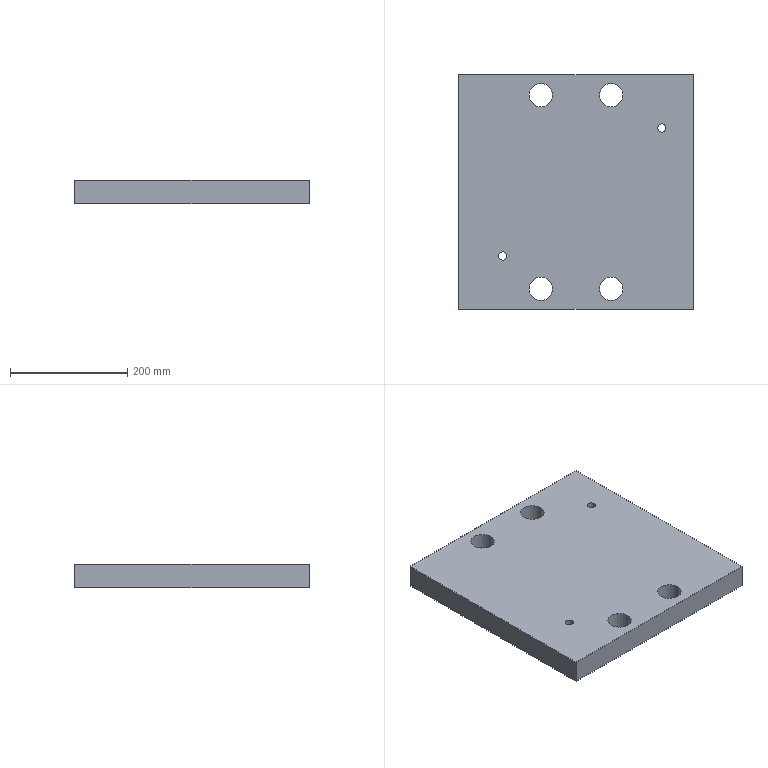Component | NX | LOCATING_BASE_PLATE | 1 solid | 12 faces | box 400 x 400 x 40 mm | volume 6186623 mm3 | plane 6 | cylinder 6 | commonest cylinder face diameters 40 x4 14 x2
STEP:
#1=CARTESIAN_POINT('',(0.,0.,0.));
#2=DIRECTION('',(0.,0.,1.));
#3=DIRECTION('',(1.,0.,0.));
#4=AXIS2_PLACEMENT_3D('',#1,#2,#3);
#5=CARTESIAN_POINT('',(-40.,165.,90.));
#6=VERTEX_POINT('',#5);
#7=CARTESIAN_POINT('',(-60.,165.,90.));
#8=DIRECTION('',(0.,0.,-1.));
#9=DIRECTION('',(1.,0.,0.));
#10=AXIS2_PLACEMENT_3D('',#7,#8,#9);
#11=CIRCLE('',#10,20.);
#12=CARTESIAN_POINT('',(0.,-0.,90.));
#13=DIRECTION('',(0.,0.,1.));
#14=DIRECTION('',(1.,0.,0.));
#15=AXIS2_PLACEMENT_3D('',#12,#13,#14);
#16=PLANE('',#15);
#17=CARTESIAN_POINT('',(-40.,165.));
#18=CARTESIAN_POINT('',(-40.,130.359));
#19=CARTESIAN_POINT('',(-70.,147.679));
#20=CARTESIAN_POINT('',(-100.,165.));
#21=CARTESIAN_POINT('',(-70.,182.321));
#22=CARTESIAN_POINT('',(-40.,199.641));
#23=CARTESIAN_POINT('',(-40.,165.));
#24=(BOUNDED_CURVE()B_SPLINE_CURVE(2,(#17,#18,#19,#20,#21,#22,#23),.UNSPECIFIED.,.T.,.F.)B_SPLINE_CURVE_WITH_KNOTS((1,2,2,2,2,1),(-2.094,0.,2.094,4.189,6.283,8.378),.UNSPECIFIED.)CURVE()GEOMETRIC_REPRESENTATION_ITEM()RATIONAL_B_SPLINE_CURVE((1.,0.5,1.,0.5,1.,0.5,1.))REPRESENTATION_ITEM(''));
#25=(GEOMETRIC_REPRESENTATION_CONTEXT(2)PARAMETRIC_REPRESENTATION_CONTEXT()REPRESENTATION_CONTEXT('',''));
#26=DEFINITIONAL_REPRESENTATION('',(#24),#25);
#27=PCURVE('',#16,#26);
#28=CARTESIAN_POINT('',(-60.,165.,40.));
#29=DIRECTION('',(0.,0.,1.));
#30=DIRECTION('',(1.,0.,0.));
#31=AXIS2_PLACEMENT_3D('',#28,#29,#30);
#32=CYLINDRICAL_SURFACE('',#31,20.);
#33=CARTESIAN_POINT('',(6.283,50.));
#34=DIRECTION('',(-1.,0.));
#35=VECTOR('',#34,1.);
#36=LINE('',#33,#35);
#37=(GEOMETRIC_REPRESENTATION_CONTEXT(2)PARAMETRIC_REPRESENTATION_CONTEXT()REPRESENTATION_CONTEXT('',''));
#38=DEFINITIONAL_REPRESENTATION('',(#36),#37);
#39=PCURVE('',#32,#38);
#40=SURFACE_CURVE('',#11,(#27,#39),.PCURVE_S1.);
#41=EDGE_CURVE('',#6,#6,#40,.T.);
#42=ORIENTED_EDGE('',*,*,#41,.T.);
#43=EDGE_LOOP('',(#42));
#44=FACE_BOUND('',#43,.T.);
#45=CARTESIAN_POINT('',(40.,165.,90.));
#46=VERTEX_POINT('',#45);
#47=CARTESIAN_POINT('',(80.,165.,90.));
#48=VERTEX_POINT('',#47);
#49=CARTESIAN_POINT('',(60.,165.,90.));
#50=DIRECTION('',(0.,0.,1.));
#51=DIRECTION('',(-1.,0.,0.));
#52=AXIS2_PLACEMENT_3D('',#49,#50,#51);
#53=CIRCLE('',#52,20.);
#54=CARTESIAN_POINT('',(60.,165.));
#55=DIRECTION('',(-1.,0.));
#56=AXIS2_PLACEMENT_2D('',#54,#55);
#57=CIRCLE('',#56,20.);
#58=(GEOMETRIC_REPRESENTATION_CONTEXT(2)PARAMETRIC_REPRESENTATION_CONTEXT()REPRESENTATION_CONTEXT('',''));
#59=DEFINITIONAL_REPRESENTATION('',(#57),#58);
#60=PCURVE('',#16,#59);
#61=CARTESIAN_POINT('',(60.,165.,40.));
#62=DIRECTION('',(0.,0.,1.));
#63=DIRECTION('',(1.,0.,0.));
#64=AXIS2_PLACEMENT_3D('',#61,#62,#63);
#65=CYLINDRICAL_SURFACE('',#64,20.);
#66=CARTESIAN_POINT('',(3.142,50.));
#67=DIRECTION('',(1.,0.));
#68=VECTOR('',#67,1.);
#69=LINE('',#66,#68);
#70=(GEOMETRIC_REPRESENTATION_CONTEXT(2)PARAMETRIC_REPRESENTATION_CONTEXT()REPRESENTATION_CONTEXT('',''));
#71=DEFINITIONAL_REPRESENTATION('',(#69),#70);
#72=PCURVE('',#65,#71);
#73=SURFACE_CURVE('',#53,(#60,#72),.PCURVE_S1.);
#74=EDGE_CURVE('',#46,#48,#73,.T.);
#75=ORIENTED_EDGE('',*,*,#74,.F.);
#76=CARTESIAN_POINT('',(60.,165.,90.));
#77=DIRECTION('',(0.,0.,1.));
#78=DIRECTION('',(-1.,0.,0.));
#79=AXIS2_PLACEMENT_3D('',#76,#77,#78);
#80=CIRCLE('',#79,20.);
#81=CARTESIAN_POINT('',(60.,165.));
#82=DIRECTION('',(-1.,0.));
#83=AXIS2_PLACEMENT_2D('',#81,#82);
#84=CIRCLE('',#83,20.);
#85=(GEOMETRIC_REPRESENTATION_CONTEXT(2)PARAMETRIC_REPRESENTATION_CONTEXT()REPRESENTATION_CONTEXT('',''));
#86=DEFINITIONAL_REPRESENTATION('',(#84),#85);
#87=PCURVE('',#16,#86);
#88=CARTESIAN_POINT('',(-3.142,50.));
#89=DIRECTION('',(1.,0.));
#90=VECTOR('',#89,1.);
#91=LINE('',#88,#90);
#92=(GEOMETRIC_REPRESENTATION_CONTEXT(2)PARAMETRIC_REPRESENTATION_CONTEXT()REPRESENTATION_CONTEXT('',''));
#93=DEFINITIONAL_REPRESENTATION('',(#91),#92);
#94=PCURVE('',#65,#93);
#95=SURFACE_CURVE('',#80,(#87,#94),.PCURVE_S1.);
#96=EDGE_CURVE('',#48,#46,#95,.T.);
#97=ORIENTED_EDGE('',*,*,#96,.F.);
#98=EDGE_LOOP('',(#75,#97));
#99=FACE_BOUND('',#98,.T.);
#100=CARTESIAN_POINT('',(153.,109.,90.));
#101=VERTEX_POINT('',#100);
#102=CARTESIAN_POINT('',(146.,109.,90.));
#103=DIRECTION('',(0.,0.,1.));
#104=DIRECTION('',(1.,0.,0.));
#105=AXIS2_PLACEMENT_3D('',#102,#103,#104);
#106=CIRCLE('',#105,7.);
#107=CARTESIAN_POINT('',(146.,109.));
#108=DIRECTION('',(1.,0.));
#109=AXIS2_PLACEMENT_2D('',#107,#108);
#110=CIRCLE('',#109,7.);
#111=(GEOMETRIC_REPRESENTATION_CONTEXT(2)PARAMETRIC_REPRESENTATION_CONTEXT()REPRESENTATION_CONTEXT('',''));
#112=DEFINITIONAL_REPRESENTATION('',(#110),#111);
#113=PCURVE('',#16,#112);
#114=CARTESIAN_POINT('',(146.,109.,50.));
#115=DIRECTION('',(0.,0.,1.));
#116=DIRECTION('',(1.,0.,0.));
#117=AXIS2_PLACEMENT_3D('',#114,#115,#116);
#118=CYLINDRICAL_SURFACE('',#117,7.);
#119=CARTESIAN_POINT('',(0.,40.));
#120=DIRECTION('',(1.,0.));
#121=VECTOR('',#120,1.);
#122=LINE('',#119,#121);
#123=(GEOMETRIC_REPRESENTATION_CONTEXT(2)PARAMETRIC_REPRESENTATION_CONTEXT()REPRESENTATION_CONTEXT('',''));
#124=DEFINITIONAL_REPRESENTATION('',(#122),#123);
#125=PCURVE('',#118,#124);
#126=SURFACE_CURVE('',#106,(#113,#125),.PCURVE_S1.);
#127=EDGE_CURVE('',#101,#101,#126,.T.);
#128=ORIENTED_EDGE('',*,*,#127,.F.);
#129=EDGE_LOOP('',(#128));
#130=FACE_BOUND('',#129,.T.);
#131=CARTESIAN_POINT('',(-118.,-109.,90.));
#132=VERTEX_POINT('',#131);
#133=CARTESIAN_POINT('',(-125.,-109.,90.));
#134=DIRECTION('',(0.,0.,1.));
#135=DIRECTION('',(1.,0.,0.));
#136=AXIS2_PLACEMENT_3D('',#133,#134,#135);
#137=CIRCLE('',#136,7.);
#138=CARTESIAN_POINT('',(-125.,-109.));
#139=DIRECTION('',(1.,0.));
#140=AXIS2_PLACEMENT_2D('',#138,#139);
#141=CIRCLE('',#140,7.);
#142=(GEOMETRIC_REPRESENTATION_CONTEXT(2)PARAMETRIC_REPRESENTATION_CONTEXT()REPRESENTATION_CONTEXT('',''));
#143=DEFINITIONAL_REPRESENTATION('',(#141),#142);
#144=PCURVE('',#16,#143);
#145=CARTESIAN_POINT('',(-125.,-109.,50.));
#146=DIRECTION('',(0.,0.,1.));
#147=DIRECTION('',(1.,0.,0.));
#148=AXIS2_PLACEMENT_3D('',#145,#146,#147);
#149=CYLINDRICAL_SURFACE('',#148,7.);
#150=CARTESIAN_POINT('',(0.,40.));
#151=DIRECTION('',(1.,0.));
#152=VECTOR('',#151,1.);
#153=LINE('',#150,#152);
#154=(GEOMETRIC_REPRESENTATION_CONTEXT(2)PARAMETRIC_REPRESENTATION_CONTEXT()REPRESENTATION_CONTEXT('',''));
#155=DEFINITIONAL_REPRESENTATION('',(#153),#154);
#156=PCURVE('',#149,#155);
#157=SURFACE_CURVE('',#137,(#144,#156),.PCURVE_S1.);
#158=EDGE_CURVE('',#132,#132,#157,.T.);
#159=ORIENTED_EDGE('',*,*,#158,.F.);
#160=EDGE_LOOP('',(#159));
#161=FACE_BOUND('',#160,.T.);
#162=CARTESIAN_POINT('',(-200.,200.,90.));
#163=VERTEX_POINT('',#162);
#164=CARTESIAN_POINT('',(-200.,-200.,90.));
#165=VERTEX_POINT('',#164);
#166=CARTESIAN_POINT('',(-200.,200.,90.));
#167=DIRECTION('',(0.,-1.,0.));
#168=VECTOR('',#167,1.);
#169=LINE('',#166,#168);
#170=CARTESIAN_POINT('',(-200.,200.));
#171=DIRECTION('',(0.,-1.));
#172=VECTOR('',#171,1.);
#173=LINE('',#170,#172);
#174=(GEOMETRIC_REPRESENTATION_CONTEXT(2)PARAMETRIC_REPRESENTATION_CONTEXT()REPRESENTATION_CONTEXT('',''));
#175=DEFINITIONAL_REPRESENTATION('',(#173),#174);
#176=PCURVE('',#16,#175);
#177=CARTESIAN_POINT('',(-200.,200.,90.));
#178=DIRECTION('',(1.,0.,0.));
#179=DIRECTION('',(0.,0.,-1.));
#180=AXIS2_PLACEMENT_3D('',#177,#178,#179);
#181=PLANE('',#180);
#182=CARTESIAN_POINT('',(0.,0.));
#183=DIRECTION('',(0.,-1.));
#184=VECTOR('',#183,1.);
#185=LINE('',#182,#184);
#186=(GEOMETRIC_REPRESENTATION_CONTEXT(2)PARAMETRIC_REPRESENTATION_CONTEXT()REPRESENTATION_CONTEXT('',''));
#187=DEFINITIONAL_REPRESENTATION('',(#185),#186);
#188=PCURVE('',#181,#187);
#189=SURFACE_CURVE('',#169,(#176,#188),.PCURVE_S1.);
#190=EDGE_CURVE('',#163,#165,#189,.T.);
#191=ORIENTED_EDGE('',*,*,#190,.T.);
#192=CARTESIAN_POINT('',(200.,-200.,90.));
#193=VERTEX_POINT('',#192);
#194=CARTESIAN_POINT('',(-200.,-200.,90.));
#195=DIRECTION('',(1.,0.,0.));
#196=VECTOR('',#195,1.);
#197=LINE('',#194,#196);
#198=CARTESIAN_POINT('',(-200.,-200.));
#199=DIRECTION('',(1.,0.));
#200=VECTOR('',#199,1.);
#201=LINE('',#198,#200);
#202=(GEOMETRIC_REPRESENTATION_CONTEXT(2)PARAMETRIC_REPRESENTATION_CONTEXT()REPRESENTATION_CONTEXT('',''));
#203=DEFINITIONAL_REPRESENTATION('',(#201),#202);
#204=PCURVE('',#16,#203);
#205=CARTESIAN_POINT('',(-200.,-200.,90.));
#206=DIRECTION('',(0.,1.,0.));
#207=DIRECTION('',(0.,0.,1.));
#208=AXIS2_PLACEMENT_3D('',#205,#206,#207);
#209=PLANE('',#208);
#210=CARTESIAN_POINT('',(0.,0.));
#211=DIRECTION('',(0.,1.));
#212=VECTOR('',#211,1.);
#213=LINE('',#210,#212);
#214=(GEOMETRIC_REPRESENTATION_CONTEXT(2)PARAMETRIC_REPRESENTATION_CONTEXT()REPRESENTATION_CONTEXT('',''));
#215=DEFINITIONAL_REPRESENTATION('',(#213),#214);
#216=PCURVE('',#209,#215);
#217=SURFACE_CURVE('',#197,(#204,#216),.PCURVE_S1.);
#218=EDGE_CURVE('',#165,#193,#217,.T.);
#219=ORIENTED_EDGE('',*,*,#218,.T.);
#220=CARTESIAN_POINT('',(200.,200.,90.));
#221=VERTEX_POINT('',#220);
#222=CARTESIAN_POINT('',(200.,-200.,90.));
#223=DIRECTION('',(0.,1.,0.));
#224=VECTOR('',#223,1.);
#225=LINE('',#222,#224);
#226=CARTESIAN_POINT('',(200.,-200.));
#227=DIRECTION('',(0.,1.));
#228=VECTOR('',#227,1.);
#229=LINE('',#226,#228);
#230=(GEOMETRIC_REPRESENTATION_CONTEXT(2)PARAMETRIC_REPRESENTATION_CONTEXT()REPRESENTATION_CONTEXT('',''));
#231=DEFINITIONAL_REPRESENTATION('',(#229),#230);
#232=PCURVE('',#16,#231);
#233=CARTESIAN_POINT('',(200.,-200.,90.));
#234=DIRECTION('',(-1.,0.,0.));
#235=DIRECTION('',(0.,0.,1.));
#236=AXIS2_PLACEMENT_3D('',#233,#234,#235);
#237=PLANE('',#236);
#238=CARTESIAN_POINT('',(0.,0.));
#239=DIRECTION('',(0.,1.));
#240=VECTOR('',#239,1.);
#241=LINE('',#238,#240);
#242=(GEOMETRIC_REPRESENTATION_CONTEXT(2)PARAMETRIC_REPRESENTATION_CONTEXT()REPRESENTATION_CONTEXT('',''));
#243=DEFINITIONAL_REPRESENTATION('',(#241),#242);
#244=PCURVE('',#237,#243);
#245=SURFACE_CURVE('',#225,(#232,#244),.PCURVE_S1.);
#246=EDGE_CURVE('',#193,#221,#245,.T.);
#247=ORIENTED_EDGE('',*,*,#246,.T.);
#248=CARTESIAN_POINT('',(200.,200.,90.));
#249=DIRECTION('',(-1.,0.,0.));
#250=VECTOR('',#249,1.);
#251=LINE('',#248,#250);
#252=CARTESIAN_POINT('',(200.,200.));
#253=DIRECTION('',(-1.,0.));
#254=VECTOR('',#253,1.);
#255=LINE('',#252,#254);
#256=(GEOMETRIC_REPRESENTATION_CONTEXT(2)PARAMETRIC_REPRESENTATION_CONTEXT()REPRESENTATION_CONTEXT('',''));
#257=DEFINITIONAL_REPRESENTATION('',(#255),#256);
#258=PCURVE('',#16,#257);
#259=CARTESIAN_POINT('',(200.,200.,90.));
#260=DIRECTION('',(0.,-1.,0.));
#261=DIRECTION('',(0.,0.,-1.));
#262=AXIS2_PLACEMENT_3D('',#259,#260,#261);
#263=PLANE('',#262);
#264=CARTESIAN_POINT('',(0.,0.));
#265=DIRECTION('',(0.,-1.));
#266=VECTOR('',#265,1.);
#267=LINE('',#264,#266);
#268=(GEOMETRIC_REPRESENTATION_CONTEXT(2)PARAMETRIC_REPRESENTATION_CONTEXT()REPRESENTATION_CONTEXT('',''));
#269=DEFINITIONAL_REPRESENTATION('',(#267),#268);
#270=PCURVE('',#263,#269);
#271=SURFACE_CURVE('',#251,(#258,#270),.PCURVE_S1.);
#272=EDGE_CURVE('',#221,#163,#271,.T.);
#273=ORIENTED_EDGE('',*,*,#272,.T.);
#274=EDGE_LOOP('',(#191,#219,#247,#273));
#275=FACE_BOUND('',#274,.T.);
#276=CARTESIAN_POINT('',(-40.,-165.,90.));
#277=VERTEX_POINT('',#276);
#278=CARTESIAN_POINT('',(-60.,-165.,90.));
#279=DIRECTION('',(0.,0.,1.));
#280=DIRECTION('',(1.,0.,0.));
#281=AXIS2_PLACEMENT_3D('',#278,#279,#280);
#282=CIRCLE('',#281,20.);
#283=CARTESIAN_POINT('',(-60.,-165.));
#284=DIRECTION('',(1.,0.));
#285=AXIS2_PLACEMENT_2D('',#283,#284);
#286=CIRCLE('',#285,20.);
#287=(GEOMETRIC_REPRESENTATION_CONTEXT(2)PARAMETRIC_REPRESENTATION_CONTEXT()REPRESENTATION_CONTEXT('',''));
#288=DEFINITIONAL_REPRESENTATION('',(#286),#287);
#289=PCURVE('',#16,#288);
#290=CARTESIAN_POINT('',(-60.,-165.,40.));
#291=DIRECTION('',(0.,0.,1.));
#292=DIRECTION('',(1.,0.,0.));
#293=AXIS2_PLACEMENT_3D('',#290,#291,#292);
#294=CYLINDRICAL_SURFACE('',#293,20.);
#295=CARTESIAN_POINT('',(0.,50.));
#296=DIRECTION('',(1.,0.));
#297=VECTOR('',#296,1.);
#298=LINE('',#295,#297);
#299=(GEOMETRIC_REPRESENTATION_CONTEXT(2)PARAMETRIC_REPRESENTATION_CONTEXT()REPRESENTATION_CONTEXT('',''));
#300=DEFINITIONAL_REPRESENTATION('',(#298),#299);
#301=PCURVE('',#294,#300);
#302=SURFACE_CURVE('',#282,(#289,#301),.PCURVE_S1.);
#303=EDGE_CURVE('',#277,#277,#302,.T.);
#304=ORIENTED_EDGE('',*,*,#303,.F.);
#305=EDGE_LOOP('',(#304));
#306=FACE_BOUND('',#305,.T.);
#307=CARTESIAN_POINT('',(40.,-165.,90.));
#308=VERTEX_POINT('',#307);
#309=CARTESIAN_POINT('',(80.,-165.,90.));
#310=VERTEX_POINT('',#309);
#311=CARTESIAN_POINT('',(60.,-165.,90.));
#312=DIRECTION('',(0.,0.,-1.));
#313=DIRECTION('',(-1.,0.,0.));
#314=AXIS2_PLACEMENT_3D('',#311,#312,#313);
#315=CIRCLE('',#314,20.);
#316=CARTESIAN_POINT('',(40.,-165.));
#317=CARTESIAN_POINT('',(40.,-130.359));
#318=CARTESIAN_POINT('',(70.,-147.679));
#319=CARTESIAN_POINT('',(100.,-165.));
#320=CARTESIAN_POINT('',(70.,-182.321));
#321=CARTESIAN_POINT('',(40.,-199.641));
#322=CARTESIAN_POINT('',(40.,-165.));
#323=(BOUNDED_CURVE()B_SPLINE_CURVE(2,(#316,#317,#318,#319,#320,#321,#322),.UNSPECIFIED.,.T.,.F.)B_SPLINE_CURVE_WITH_KNOTS((1,2,2,2,2,1),(-2.094,0.,2.094,4.189,6.283,8.378),.UNSPECIFIED.)CURVE()GEOMETRIC_REPRESENTATION_ITEM()RATIONAL_B_SPLINE_CURVE((1.,0.5,1.,0.5,1.,0.5,1.))REPRESENTATION_ITEM(''));
#324=(GEOMETRIC_REPRESENTATION_CONTEXT(2)PARAMETRIC_REPRESENTATION_CONTEXT()REPRESENTATION_CONTEXT('',''));
#325=DEFINITIONAL_REPRESENTATION('',(#323),#324);
#326=PCURVE('',#16,#325);
#327=CARTESIAN_POINT('',(60.,-165.,40.));
#328=DIRECTION('',(0.,0.,1.));
#329=DIRECTION('',(1.,0.,0.));
#330=AXIS2_PLACEMENT_3D('',#327,#328,#329);
#331=CYLINDRICAL_SURFACE('',#330,20.);
#332=CARTESIAN_POINT('',(3.142,50.));
#333=DIRECTION('',(-1.,0.));
#334=VECTOR('',#333,1.);
#335=LINE('',#332,#334);
#336=(GEOMETRIC_REPRESENTATION_CONTEXT(2)PARAMETRIC_REPRESENTATION_CONTEXT()REPRESENTATION_CONTEXT('',''));
#337=DEFINITIONAL_REPRESENTATION('',(#335),#336);
#338=PCURVE('',#331,#337);
#339=SURFACE_CURVE('',#315,(#326,#338),.PCURVE_S1.);
#340=EDGE_CURVE('',#308,#310,#339,.T.);
#341=ORIENTED_EDGE('',*,*,#340,.T.);
#342=CARTESIAN_POINT('',(60.,-165.,90.));
#343=DIRECTION('',(0.,0.,-1.));
#344=DIRECTION('',(-1.,0.,0.));
#345=AXIS2_PLACEMENT_3D('',#342,#343,#344);
#346=CIRCLE('',#345,20.);
#347=CARTESIAN_POINT('',(40.,-165.));
#348=CARTESIAN_POINT('',(40.,-130.359));
#349=CARTESIAN_POINT('',(70.,-147.679));
#350=CARTESIAN_POINT('',(100.,-165.));
#351=CARTESIAN_POINT('',(70.,-182.321));
#352=CARTESIAN_POINT('',(40.,-199.641));
#353=CARTESIAN_POINT('',(40.,-165.));
#354=(BOUNDED_CURVE()B_SPLINE_CURVE(2,(#347,#348,#349,#350,#351,#352,#353),.UNSPECIFIED.,.T.,.F.)B_SPLINE_CURVE_WITH_KNOTS((1,2,2,2,2,1),(-2.094,0.,2.094,4.189,6.283,8.378),.UNSPECIFIED.)CURVE()GEOMETRIC_REPRESENTATION_ITEM()RATIONAL_B_SPLINE_CURVE((1.,0.5,1.,0.5,1.,0.5,1.))REPRESENTATION_ITEM(''));
#355=(GEOMETRIC_REPRESENTATION_CONTEXT(2)PARAMETRIC_REPRESENTATION_CONTEXT()REPRESENTATION_CONTEXT('',''));
#356=DEFINITIONAL_REPRESENTATION('',(#354),#355);
#357=PCURVE('',#16,#356);
#358=CARTESIAN_POINT('',(9.425,50.));
#359=DIRECTION('',(-1.,0.));
#360=VECTOR('',#359,1.);
#361=LINE('',#358,#360);
#362=(GEOMETRIC_REPRESENTATION_CONTEXT(2)PARAMETRIC_REPRESENTATION_CONTEXT()REPRESENTATION_CONTEXT('',''));
#363=DEFINITIONAL_REPRESENTATION('',(#361),#362);
#364=PCURVE('',#331,#363);
#365=SURFACE_CURVE('',#346,(#357,#364),.PCURVE_S1.);
#366=EDGE_CURVE('',#310,#308,#365,.T.);
#367=ORIENTED_EDGE('',*,*,#366,.T.);
#368=EDGE_LOOP('',(#341,#367));
#369=FACE_BOUND('',#368,.T.);
#370=ADVANCED_FACE('',(#44,#99,#130,#161,#275,#306,#369),#16,.T.);
#371=CARTESIAN_POINT('',(-40.,-165.,50.));
#372=VERTEX_POINT('',#371);
#373=CARTESIAN_POINT('',(-60.,-165.,50.));
#374=DIRECTION('',(0.,0.,1.));
#375=DIRECTION('',(1.,0.,0.));
#376=AXIS2_PLACEMENT_3D('',#373,#374,#375);
#377=CIRCLE('',#376,20.);
#378=CARTESIAN_POINT('',(0.,-0.,50.));
#379=DIRECTION('',(0.,0.,1.));
#380=DIRECTION('',(1.,0.,0.));
#381=AXIS2_PLACEMENT_3D('',#378,#379,#380);
#382=PLANE('',#381);
#383=CARTESIAN_POINT('',(-60.,-165.));
#384=DIRECTION('',(1.,0.));
#385=AXIS2_PLACEMENT_2D('',#383,#384);
#386=CIRCLE('',#385,20.);
#387=(GEOMETRIC_REPRESENTATION_CONTEXT(2)PARAMETRIC_REPRESENTATION_CONTEXT()REPRESENTATION_CONTEXT('',''));
#388=DEFINITIONAL_REPRESENTATION('',(#386),#387);
#389=PCURVE('',#382,#388);
#390=CARTESIAN_POINT('',(0.,10.));
#391=DIRECTION('',(1.,0.));
#392=VECTOR('',#391,1.);
#393=LINE('',#390,#392);
#394=(GEOMETRIC_REPRESENTATION_CONTEXT(2)PARAMETRIC_REPRESENTATION_CONTEXT()REPRESENTATION_CONTEXT('',''));
#395=DEFINITIONAL_REPRESENTATION('',(#393),#394);
#396=PCURVE('',#294,#395);
#397=SURFACE_CURVE('',#377,(#389,#396),.PCURVE_S1.);
#398=EDGE_CURVE('',#372,#372,#397,.T.);
#399=ORIENTED_EDGE('',*,*,#398,.T.);
#400=EDGE_LOOP('',(#399));
#401=FACE_BOUND('',#400,.T.);
#402=CARTESIAN_POINT('',(80.,165.,50.));
#403=VERTEX_POINT('',#402);
#404=CARTESIAN_POINT('',(60.,165.,50.));
#405=DIRECTION('',(0.,0.,1.));
#406=DIRECTION('',(1.,0.,0.));
#407=AXIS2_PLACEMENT_3D('',#404,#405,#406);
#408=CIRCLE('',#407,20.);
#409=CARTESIAN_POINT('',(60.,165.));
#410=DIRECTION('',(1.,0.));
#411=AXIS2_PLACEMENT_2D('',#409,#410);
#412=CIRCLE('',#411,20.);
#413=(GEOMETRIC_REPRESENTATION_CONTEXT(2)PARAMETRIC_REPRESENTATION_CONTEXT()REPRESENTATION_CONTEXT('',''));
#414=DEFINITIONAL_REPRESENTATION('',(#412),#413);
#415=PCURVE('',#382,#414);
#416=CARTESIAN_POINT('',(0.,10.));
#417=DIRECTION('',(1.,0.));
#418=VECTOR('',#417,1.);
#419=LINE('',#416,#418);
#420=(GEOMETRIC_REPRESENTATION_CONTEXT(2)PARAMETRIC_REPRESENTATION_CONTEXT()REPRESENTATION_CONTEXT('',''));
#421=DEFINITIONAL_REPRESENTATION('',(#419),#420);
#422=PCURVE('',#65,#421);
#423=SURFACE_CURVE('',#408,(#415,#422),.PCURVE_S1.);
#424=EDGE_CURVE('',#403,#403,#423,.T.);
#425=ORIENTED_EDGE('',*,*,#424,.T.);
#426=EDGE_LOOP('',(#425));
#427=FACE_BOUND('',#426,.T.);
#428=CARTESIAN_POINT('',(153.,109.,50.));
#429=VERTEX_POINT('',#428);
#430=CARTESIAN_POINT('',(146.,109.,50.));
#431=DIRECTION('',(0.,0.,1.));
#432=DIRECTION('',(1.,0.,0.));
#433=AXIS2_PLACEMENT_3D('',#430,#431,#432);
#434=CIRCLE('',#433,7.);
#435=CARTESIAN_POINT('',(146.,109.));
#436=DIRECTION('',(1.,0.));
#437=AXIS2_PLACEMENT_2D('',#435,#436);
#438=CIRCLE('',#437,7.);
#439=(GEOMETRIC_REPRESENTATION_CONTEXT(2)PARAMETRIC_REPRESENTATION_CONTEXT()REPRESENTATION_CONTEXT('',''));
#440=DEFINITIONAL_REPRESENTATION('',(#438),#439);
#441=PCURVE('',#382,#440);
#442=CARTESIAN_POINT('',(0.,0.));
#443=DIRECTION('',(1.,0.));
#444=VECTOR('',#443,1.);
#445=LINE('',#442,#444);
#446=(GEOMETRIC_REPRESENTATION_CONTEXT(2)PARAMETRIC_REPRESENTATION_CONTEXT()REPRESENTATION_CONTEXT('',''));
#447=DEFINITIONAL_REPRESENTATION('',(#445),#446);
#448=PCURVE('',#118,#447);
#449=SURFACE_CURVE('',#434,(#441,#448),.PCURVE_S1.);
#450=EDGE_CURVE('',#429,#429,#449,.T.);
#451=ORIENTED_EDGE('',*,*,#450,.T.);
#452=EDGE_LOOP('',(#451));
#453=FACE_BOUND('',#452,.T.);
#454=CARTESIAN_POINT('',(-118.,-109.,50.));
#455=VERTEX_POINT('',#454);
#456=CARTESIAN_POINT('',(-125.,-109.,50.));
#457=DIRECTION('',(0.,0.,1.));
#458=DIRECTION('',(1.,0.,0.));
#459=AXIS2_PLACEMENT_3D('',#456,#457,#458);
#460=CIRCLE('',#459,7.);
#461=CARTESIAN_POINT('',(-125.,-109.));
#462=DIRECTION('',(1.,0.));
#463=AXIS2_PLACEMENT_2D('',#461,#462);
#464=CIRCLE('',#463,7.);
#465=(GEOMETRIC_REPRESENTATION_CONTEXT(2)PARAMETRIC_REPRESENTATION_CONTEXT()REPRESENTATION_CONTEXT('',''));
#466=DEFINITIONAL_REPRESENTATION('',(#464),#465);
#467=PCURVE('',#382,#466);
#468=CARTESIAN_POINT('',(0.,0.));
#469=DIRECTION('',(1.,0.));
#470=VECTOR('',#469,1.);
#471=LINE('',#468,#470);
#472=(GEOMETRIC_REPRESENTATION_CONTEXT(2)PARAMETRIC_REPRESENTATION_CONTEXT()REPRESENTATION_CONTEXT('',''));
#473=DEFINITIONAL_REPRESENTATION('',(#471),#472);
#474=PCURVE('',#149,#473);
#475=SURFACE_CURVE('',#460,(#467,#474),.PCURVE_S1.);
#476=EDGE_CURVE('',#455,#455,#475,.T.);
#477=ORIENTED_EDGE('',*,*,#476,.T.);
#478=EDGE_LOOP('',(#477));
#479=FACE_BOUND('',#478,.T.);
#480=CARTESIAN_POINT('',(-200.,200.,50.));
#481=VERTEX_POINT('',#480);
#482=CARTESIAN_POINT('',(-200.,-200.,50.));
#483=VERTEX_POINT('',#482);
#484=CARTESIAN_POINT('',(-200.,200.,50.));
#485=DIRECTION('',(0.,-1.,0.));
#486=VECTOR('',#485,1.);
#487=LINE('',#484,#486);
#488=CARTESIAN_POINT('',(-200.,200.));
#489=DIRECTION('',(0.,-1.));
#490=VECTOR('',#489,1.);
#491=LINE('',#488,#490);
#492=(GEOMETRIC_REPRESENTATION_CONTEXT(2)PARAMETRIC_REPRESENTATION_CONTEXT()REPRESENTATION_CONTEXT('',''));
#493=DEFINITIONAL_REPRESENTATION('',(#491),#492);
#494=PCURVE('',#382,#493);
#495=CARTESIAN_POINT('',(40.,0.));
#496=DIRECTION('',(0.,-1.));
#497=VECTOR('',#496,1.);
#498=LINE('',#495,#497);
#499=(GEOMETRIC_REPRESENTATION_CONTEXT(2)PARAMETRIC_REPRESENTATION_CONTEXT()REPRESENTATION_CONTEXT('',''));
#500=DEFINITIONAL_REPRESENTATION('',(#498),#499);
#501=PCURVE('',#181,#500);
#502=SURFACE_CURVE('',#487,(#494,#501),.PCURVE_S1.);
#503=EDGE_CURVE('',#481,#483,#502,.T.);
#504=ORIENTED_EDGE('',*,*,#503,.F.);
#505=CARTESIAN_POINT('',(200.,200.,50.));
#506=VERTEX_POINT('',#505);
#507=CARTESIAN_POINT('',(200.,200.,50.));
#508=DIRECTION('',(-1.,0.,0.));
#509=VECTOR('',#508,1.);
#510=LINE('',#507,#509);
#511=CARTESIAN_POINT('',(200.,200.));
#512=DIRECTION('',(-1.,0.));
#513=VECTOR('',#512,1.);
#514=LINE('',#511,#513);
#515=(GEOMETRIC_REPRESENTATION_CONTEXT(2)PARAMETRIC_REPRESENTATION_CONTEXT()REPRESENTATION_CONTEXT('',''));
#516=DEFINITIONAL_REPRESENTATION('',(#514),#515);
#517=PCURVE('',#382,#516);
#518=CARTESIAN_POINT('',(40.,0.));
#519=DIRECTION('',(0.,-1.));
#520=VECTOR('',#519,1.);
#521=LINE('',#518,#520);
#522=(GEOMETRIC_REPRESENTATION_CONTEXT(2)PARAMETRIC_REPRESENTATION_CONTEXT()REPRESENTATION_CONTEXT('',''));
#523=DEFINITIONAL_REPRESENTATION('',(#521),#522);
#524=PCURVE('',#263,#523);
#525=SURFACE_CURVE('',#510,(#517,#524),.PCURVE_S1.);
#526=EDGE_CURVE('',#506,#481,#525,.T.);
#527=ORIENTED_EDGE('',*,*,#526,.F.);
#528=CARTESIAN_POINT('',(200.,-200.,50.));
#529=VERTEX_POINT('',#528);
#530=CARTESIAN_POINT('',(200.,-200.,50.));
#531=DIRECTION('',(0.,1.,0.));
#532=VECTOR('',#531,1.);
#533=LINE('',#530,#532);
#534=CARTESIAN_POINT('',(200.,-200.));
#535=DIRECTION('',(0.,1.));
#536=VECTOR('',#535,1.);
#537=LINE('',#534,#536);
#538=(GEOMETRIC_REPRESENTATION_CONTEXT(2)PARAMETRIC_REPRESENTATION_CONTEXT()REPRESENTATION_CONTEXT('',''));
#539=DEFINITIONAL_REPRESENTATION('',(#537),#538);
#540=PCURVE('',#382,#539);
#541=CARTESIAN_POINT('',(-40.,0.));
#542=DIRECTION('',(0.,1.));
#543=VECTOR('',#542,1.);
#544=LINE('',#541,#543);
#545=(GEOMETRIC_REPRESENTATION_CONTEXT(2)PARAMETRIC_REPRESENTATION_CONTEXT()REPRESENTATION_CONTEXT('',''));
#546=DEFINITIONAL_REPRESENTATION('',(#544),#545);
#547=PCURVE('',#237,#546);
#548=SURFACE_CURVE('',#533,(#540,#547),.PCURVE_S1.);
#549=EDGE_CURVE('',#529,#506,#548,.T.);
#550=ORIENTED_EDGE('',*,*,#549,.F.);
#551=CARTESIAN_POINT('',(-200.,-200.,50.));
#552=DIRECTION('',(1.,0.,0.));
#553=VECTOR('',#552,1.);
#554=LINE('',#551,#553);
#555=CARTESIAN_POINT('',(-200.,-200.));
#556=DIRECTION('',(1.,0.));
#557=VECTOR('',#556,1.);
#558=LINE('',#555,#557);
#559=(GEOMETRIC_REPRESENTATION_CONTEXT(2)PARAMETRIC_REPRESENTATION_CONTEXT()REPRESENTATION_CONTEXT('',''));
#560=DEFINITIONAL_REPRESENTATION('',(#558),#559);
#561=PCURVE('',#382,#560);
#562=CARTESIAN_POINT('',(-40.,0.));
#563=DIRECTION('',(0.,1.));
#564=VECTOR('',#563,1.);
#565=LINE('',#562,#564);
#566=(GEOMETRIC_REPRESENTATION_CONTEXT(2)PARAMETRIC_REPRESENTATION_CONTEXT()REPRESENTATION_CONTEXT('',''));
#567=DEFINITIONAL_REPRESENTATION('',(#565),#566);
#568=PCURVE('',#209,#567);
#569=SURFACE_CURVE('',#554,(#561,#568),.PCURVE_S1.);
#570=EDGE_CURVE('',#483,#529,#569,.T.);
#571=ORIENTED_EDGE('',*,*,#570,.F.);
#572=EDGE_LOOP('',(#504,#527,#550,#571));
#573=FACE_BOUND('',#572,.T.);
#574=CARTESIAN_POINT('',(-40.,165.,50.));
#575=VERTEX_POINT('',#574);
#576=CARTESIAN_POINT('',(-60.,165.,50.));
#577=DIRECTION('',(0.,0.,-1.));
#578=DIRECTION('',(1.,0.,0.));
#579=AXIS2_PLACEMENT_3D('',#576,#577,#578);
#580=CIRCLE('',#579,20.);
#581=CARTESIAN_POINT('',(-40.,165.));
#582=CARTESIAN_POINT('',(-40.,130.359));
#583=CARTESIAN_POINT('',(-70.,147.679));
#584=CARTESIAN_POINT('',(-100.,165.));
#585=CARTESIAN_POINT('',(-70.,182.321));
#586=CARTESIAN_POINT('',(-40.,199.641));
#587=CARTESIAN_POINT('',(-40.,165.));
#588=(BOUNDED_CURVE()B_SPLINE_CURVE(2,(#581,#582,#583,#584,#585,#586,#587),.UNSPECIFIED.,.T.,.F.)B_SPLINE_CURVE_WITH_KNOTS((1,2,2,2,2,1),(-2.094,0.,2.094,4.189,6.283,8.378),.UNSPECIFIED.)CURVE()GEOMETRIC_REPRESENTATION_ITEM()RATIONAL_B_SPLINE_CURVE((1.,0.5,1.,0.5,1.,0.5,1.))REPRESENTATION_ITEM(''));
#589=(GEOMETRIC_REPRESENTATION_CONTEXT(2)PARAMETRIC_REPRESENTATION_CONTEXT()REPRESENTATION_CONTEXT('',''));
#590=DEFINITIONAL_REPRESENTATION('',(#588),#589);
#591=PCURVE('',#382,#590);
#592=CARTESIAN_POINT('',(6.283,10.));
#593=DIRECTION('',(-1.,0.));
#594=VECTOR('',#593,1.);
#595=LINE('',#592,#594);
#596=(GEOMETRIC_REPRESENTATION_CONTEXT(2)PARAMETRIC_REPRESENTATION_CONTEXT()REPRESENTATION_CONTEXT('',''));
#597=DEFINITIONAL_REPRESENTATION('',(#595),#596);
#598=PCURVE('',#32,#597);
#599=SURFACE_CURVE('',#580,(#591,#598),.PCURVE_S1.);
#600=EDGE_CURVE('',#575,#575,#599,.T.);
#601=ORIENTED_EDGE('',*,*,#600,.F.);
#602=EDGE_LOOP('',(#601));
#603=FACE_BOUND('',#602,.T.);
#604=CARTESIAN_POINT('',(80.,-165.,50.));
#605=VERTEX_POINT('',#604);
#606=CARTESIAN_POINT('',(60.,-165.,50.));
#607=DIRECTION('',(0.,0.,-1.));
#608=DIRECTION('',(1.,0.,0.));
#609=AXIS2_PLACEMENT_3D('',#606,#607,#608);
#610=CIRCLE('',#609,20.);
#611=CARTESIAN_POINT('',(80.,-165.));
#612=CARTESIAN_POINT('',(80.,-199.641));
#613=CARTESIAN_POINT('',(50.,-182.321));
#614=CARTESIAN_POINT('',(20.,-165.));
#615=CARTESIAN_POINT('',(50.,-147.679));
#616=CARTESIAN_POINT('',(80.,-130.359));
#617=CARTESIAN_POINT('',(80.,-165.));
#618=(BOUNDED_CURVE()B_SPLINE_CURVE(2,(#611,#612,#613,#614,#615,#616,#617),.UNSPECIFIED.,.T.,.F.)B_SPLINE_CURVE_WITH_KNOTS((1,2,2,2,2,1),(-2.094,0.,2.094,4.189,6.283,8.378),.UNSPECIFIED.)CURVE()GEOMETRIC_REPRESENTATION_ITEM()RATIONAL_B_SPLINE_CURVE((1.,0.5,1.,0.5,1.,0.5,1.))REPRESENTATION_ITEM(''));
#619=(GEOMETRIC_REPRESENTATION_CONTEXT(2)PARAMETRIC_REPRESENTATION_CONTEXT()REPRESENTATION_CONTEXT('',''));
#620=DEFINITIONAL_REPRESENTATION('',(#618),#619);
#621=PCURVE('',#382,#620);
#622=CARTESIAN_POINT('',(6.283,10.));
#623=DIRECTION('',(-1.,0.));
#624=VECTOR('',#623,1.);
#625=LINE('',#622,#624);
#626=(GEOMETRIC_REPRESENTATION_CONTEXT(2)PARAMETRIC_REPRESENTATION_CONTEXT()REPRESENTATION_CONTEXT('',''));
#627=DEFINITIONAL_REPRESENTATION('',(#625),#626);
#628=PCURVE('',#331,#627);
#629=SURFACE_CURVE('',#610,(#621,#628),.PCURVE_S1.);
#630=EDGE_CURVE('',#605,#605,#629,.T.);
#631=ORIENTED_EDGE('',*,*,#630,.F.);
#632=EDGE_LOOP('',(#631));
#633=FACE_BOUND('',#632,.T.);
#634=ADVANCED_FACE('',(#401,#427,#453,#479,#573,#603,#633),#382,.F.);
#635=ORIENTED_EDGE('',*,*,#503,.T.);
#636=CARTESIAN_POINT('',(-200.,-200.,90.));
#637=DIRECTION('',(0.,0.,-1.));
#638=VECTOR('',#637,1.);
#639=LINE('',#636,#638);
#640=CARTESIAN_POINT('',(0.,-400.));
#641=DIRECTION('',(1.,0.));
#642=VECTOR('',#641,1.);
#643=LINE('',#640,#642);
#644=(GEOMETRIC_REPRESENTATION_CONTEXT(2)PARAMETRIC_REPRESENTATION_CONTEXT()REPRESENTATION_CONTEXT('',''));
#645=DEFINITIONAL_REPRESENTATION('',(#643),#644);
#646=PCURVE('',#181,#645);
#647=CARTESIAN_POINT('',(0.,0.));
#648=DIRECTION('',(-1.,0.));
#649=VECTOR('',#648,1.);
#650=LINE('',#647,#649);
#651=(GEOMETRIC_REPRESENTATION_CONTEXT(2)PARAMETRIC_REPRESENTATION_CONTEXT()REPRESENTATION_CONTEXT('',''));
#652=DEFINITIONAL_REPRESENTATION('',(#650),#651);
#653=PCURVE('',#209,#652);
#654=SURFACE_CURVE('',#639,(#646,#653),.PCURVE_S1.);
#655=EDGE_CURVE('',#165,#483,#654,.T.);
#656=ORIENTED_EDGE('',*,*,#655,.F.);
#657=ORIENTED_EDGE('',*,*,#190,.F.);
#658=CARTESIAN_POINT('',(-200.,200.,90.));
#659=DIRECTION('',(0.,0.,-1.));
#660=VECTOR('',#659,1.);
#661=LINE('',#658,#660);
#662=CARTESIAN_POINT('',(0.,0.));
#663=DIRECTION('',(1.,0.));
#664=VECTOR('',#663,1.);
#665=LINE('',#662,#664);
#666=(GEOMETRIC_REPRESENTATION_CONTEXT(2)PARAMETRIC_REPRESENTATION_CONTEXT()REPRESENTATION_CONTEXT('',''));
#667=DEFINITIONAL_REPRESENTATION('',(#665),#666);
#668=PCURVE('',#181,#667);
#669=CARTESIAN_POINT('',(0.,-400.));
#670=DIRECTION('',(1.,0.));
#671=VECTOR('',#670,1.);
#672=LINE('',#669,#671);
#673=(GEOMETRIC_REPRESENTATION_CONTEXT(2)PARAMETRIC_REPRESENTATION_CONTEXT()REPRESENTATION_CONTEXT('',''));
#674=DEFINITIONAL_REPRESENTATION('',(#672),#673);
#675=PCURVE('',#263,#674);
#676=SURFACE_CURVE('',#661,(#668,#675),.PCURVE_S1.);
#677=EDGE_CURVE('',#163,#481,#676,.T.);
#678=ORIENTED_EDGE('',*,*,#677,.T.);
#679=EDGE_LOOP('',(#635,#656,#657,#678));
#680=FACE_BOUND('',#679,.T.);
#681=ADVANCED_FACE('',(#680),#181,.F.);
#682=ORIENTED_EDGE('',*,*,#570,.T.);
#683=CARTESIAN_POINT('',(200.,-200.,90.));
#684=DIRECTION('',(0.,0.,-1.));
#685=VECTOR('',#684,1.);
#686=LINE('',#683,#685);
#687=CARTESIAN_POINT('',(0.,400.));
#688=DIRECTION('',(-1.,0.));
#689=VECTOR('',#688,1.);
#690=LINE('',#687,#689);
#691=(GEOMETRIC_REPRESENTATION_CONTEXT(2)PARAMETRIC_REPRESENTATION_CONTEXT()REPRESENTATION_CONTEXT('',''));
#692=DEFINITIONAL_REPRESENTATION('',(#690),#691);
#693=PCURVE('',#209,#692);
#694=CARTESIAN_POINT('',(0.,0.));
#695=DIRECTION('',(-1.,0.));
#696=VECTOR('',#695,1.);
#697=LINE('',#694,#696);
#698=(GEOMETRIC_REPRESENTATION_CONTEXT(2)PARAMETRIC_REPRESENTATION_CONTEXT()REPRESENTATION_CONTEXT('',''));
#699=DEFINITIONAL_REPRESENTATION('',(#697),#698);
#700=PCURVE('',#237,#699);
#701=SURFACE_CURVE('',#686,(#693,#700),.PCURVE_S1.);
#702=EDGE_CURVE('',#193,#529,#701,.T.);
#703=ORIENTED_EDGE('',*,*,#702,.F.);
#704=ORIENTED_EDGE('',*,*,#218,.F.);
#705=ORIENTED_EDGE('',*,*,#655,.T.);
#706=EDGE_LOOP('',(#682,#703,#704,#705));
#707=FACE_BOUND('',#706,.T.);
#708=ADVANCED_FACE('',(#707),#209,.F.);
#709=ORIENTED_EDGE('',*,*,#549,.T.);
#710=CARTESIAN_POINT('',(200.,200.,90.));
#711=DIRECTION('',(0.,0.,-1.));
#712=VECTOR('',#711,1.);
#713=LINE('',#710,#712);
#714=CARTESIAN_POINT('',(0.,400.));
#715=DIRECTION('',(-1.,0.));
#716=VECTOR('',#715,1.);
#717=LINE('',#714,#716);
#718=(GEOMETRIC_REPRESENTATION_CONTEXT(2)PARAMETRIC_REPRESENTATION_CONTEXT()REPRESENTATION_CONTEXT('',''));
#719=DEFINITIONAL_REPRESENTATION('',(#717),#718);
#720=PCURVE('',#237,#719);
#721=CARTESIAN_POINT('',(0.,0.));
#722=DIRECTION('',(1.,0.));
#723=VECTOR('',#722,1.);
#724=LINE('',#721,#723);
#725=(GEOMETRIC_REPRESENTATION_CONTEXT(2)PARAMETRIC_REPRESENTATION_CONTEXT()REPRESENTATION_CONTEXT('',''));
#726=DEFINITIONAL_REPRESENTATION('',(#724),#725);
#727=PCURVE('',#263,#726);
#728=SURFACE_CURVE('',#713,(#720,#727),.PCURVE_S1.);
#729=EDGE_CURVE('',#221,#506,#728,.T.);
#730=ORIENTED_EDGE('',*,*,#729,.F.);
#731=ORIENTED_EDGE('',*,*,#246,.F.);
#732=ORIENTED_EDGE('',*,*,#702,.T.);
#733=EDGE_LOOP('',(#709,#730,#731,#732));
#734=FACE_BOUND('',#733,.T.);
#735=ADVANCED_FACE('',(#734),#237,.F.);
#736=ORIENTED_EDGE('',*,*,#526,.T.);
#737=ORIENTED_EDGE('',*,*,#677,.F.);
#738=ORIENTED_EDGE('',*,*,#272,.F.);
#739=ORIENTED_EDGE('',*,*,#729,.T.);
#740=EDGE_LOOP('',(#736,#737,#738,#739));
#741=FACE_BOUND('',#740,.T.);
#742=ADVANCED_FACE('',(#741),#263,.F.);
#743=ORIENTED_EDGE('',*,*,#476,.T.);
#744=CARTESIAN_POINT('',(-118.,-109.,50.));
#745=CARTESIAN_POINT('',(-118.,-109.,90.));
#746=B_SPLINE_CURVE_WITH_KNOTS('',1,(#744,#745),.UNSPECIFIED.,.F.,.F.,(2,2),(0.,40.),.PIECEWISE_BEZIER_KNOTS.);
#747=CARTESIAN_POINT('',(6.283,0.));
#748=DIRECTION('',(0.,1.));
#749=VECTOR('',#748,1.);
#750=LINE('',#747,#749);
#751=(GEOMETRIC_REPRESENTATION_CONTEXT(2)PARAMETRIC_REPRESENTATION_CONTEXT()REPRESENTATION_CONTEXT('',''));
#752=DEFINITIONAL_REPRESENTATION('',(#750),#751);
#753=PCURVE('',#149,#752);
#754=CARTESIAN_POINT('',(0.,0.));
#755=DIRECTION('',(0.,1.));
#756=VECTOR('',#755,1.);
#757=LINE('',#754,#756);
#758=(GEOMETRIC_REPRESENTATION_CONTEXT(2)PARAMETRIC_REPRESENTATION_CONTEXT()REPRESENTATION_CONTEXT('',''));
#759=DEFINITIONAL_REPRESENTATION('',(#757),#758);
#760=PCURVE('',#149,#759);
#761=SEAM_CURVE('',#746,(#753,#760),.PCURVE_S1.);
#762=EDGE_CURVE('',#455,#132,#761,.T.);
#763=ORIENTED_EDGE('',*,*,#762,.T.);
#764=ORIENTED_EDGE('',*,*,#158,.F.);
#765=ORIENTED_EDGE('',*,*,#762,.F.);
#766=EDGE_LOOP('',(#743,#763,#764,#765));
#767=FACE_BOUND('',#766,.F.);
#768=ADVANCED_FACE('',(#767),#149,.F.);
#769=ORIENTED_EDGE('',*,*,#450,.T.);
#770=CARTESIAN_POINT('',(153.,109.,50.));
#771=CARTESIAN_POINT('',(153.,109.,90.));
#772=B_SPLINE_CURVE_WITH_KNOTS('',1,(#770,#771),.UNSPECIFIED.,.F.,.F.,(2,2),(0.,40.),.PIECEWISE_BEZIER_KNOTS.);
#773=CARTESIAN_POINT('',(6.283,0.));
#774=DIRECTION('',(0.,1.));
#775=VECTOR('',#774,1.);
#776=LINE('',#773,#775);
#777=(GEOMETRIC_REPRESENTATION_CONTEXT(2)PARAMETRIC_REPRESENTATION_CONTEXT()REPRESENTATION_CONTEXT('',''));
#778=DEFINITIONAL_REPRESENTATION('',(#776),#777);
#779=PCURVE('',#118,#778);
#780=CARTESIAN_POINT('',(0.,0.));
#781=DIRECTION('',(0.,1.));
#782=VECTOR('',#781,1.);
#783=LINE('',#780,#782);
#784=(GEOMETRIC_REPRESENTATION_CONTEXT(2)PARAMETRIC_REPRESENTATION_CONTEXT()REPRESENTATION_CONTEXT('',''));
#785=DEFINITIONAL_REPRESENTATION('',(#783),#784);
#786=PCURVE('',#118,#785);
#787=SEAM_CURVE('',#772,(#779,#786),.PCURVE_S1.);
#788=EDGE_CURVE('',#429,#101,#787,.T.);
#789=ORIENTED_EDGE('',*,*,#788,.T.);
#790=ORIENTED_EDGE('',*,*,#127,.F.);
#791=ORIENTED_EDGE('',*,*,#788,.F.);
#792=EDGE_LOOP('',(#769,#789,#790,#791));
#793=FACE_BOUND('',#792,.F.);
#794=ADVANCED_FACE('',(#793),#118,.F.);
#795=ORIENTED_EDGE('',*,*,#96,.F.);
#796=CARTESIAN_POINT('',(80.,165.,50.));
#797=CARTESIAN_POINT('',(80.,165.,90.));
#798=B_SPLINE_CURVE_WITH_KNOTS('',1,(#796,#797),.UNSPECIFIED.,.F.,.F.,(2,2),(10.,50.),.PIECEWISE_BEZIER_KNOTS.);
#799=CARTESIAN_POINT('',(0.,0.));
#800=DIRECTION('',(0.,1.));
#801=VECTOR('',#800,1.);
#802=LINE('',#799,#801);
#803=(GEOMETRIC_REPRESENTATION_CONTEXT(2)PARAMETRIC_REPRESENTATION_CONTEXT()REPRESENTATION_CONTEXT('',''));
#804=DEFINITIONAL_REPRESENTATION('',(#802),#803);
#805=PCURVE('',#65,#804);
#806=CARTESIAN_POINT('',(6.283,0.));
#807=DIRECTION('',(0.,1.));
#808=VECTOR('',#807,1.);
#809=LINE('',#806,#808);
#810=(GEOMETRIC_REPRESENTATION_CONTEXT(2)PARAMETRIC_REPRESENTATION_CONTEXT()REPRESENTATION_CONTEXT('',''));
#811=DEFINITIONAL_REPRESENTATION('',(#809),#810);
#812=PCURVE('',#65,#811);
#813=SEAM_CURVE('',#798,(#805,#812),.PCURVE_S1.);
#814=EDGE_CURVE('',#403,#48,#813,.T.);
#815=ORIENTED_EDGE('',*,*,#814,.F.);
#816=ORIENTED_EDGE('',*,*,#424,.T.);
#817=ORIENTED_EDGE('',*,*,#814,.T.);
#818=ORIENTED_EDGE('',*,*,#74,.F.);
#819=EDGE_LOOP('',(#795,#815,#816,#817,#818));
#820=FACE_BOUND('',#819,.F.);
#821=ADVANCED_FACE('',(#820),#65,.F.);
#822=ORIENTED_EDGE('',*,*,#41,.T.);
#823=CARTESIAN_POINT('',(-40.,165.,50.));
#824=CARTESIAN_POINT('',(-40.,165.,90.));
#825=B_SPLINE_CURVE_WITH_KNOTS('',1,(#823,#824),.UNSPECIFIED.,.F.,.F.,(2,2),(10.,50.),.PIECEWISE_BEZIER_KNOTS.);
#826=CARTESIAN_POINT('',(0.,0.));
#827=DIRECTION('',(0.,1.));
#828=VECTOR('',#827,1.);
#829=LINE('',#826,#828);
#830=(GEOMETRIC_REPRESENTATION_CONTEXT(2)PARAMETRIC_REPRESENTATION_CONTEXT()REPRESENTATION_CONTEXT('',''));
#831=DEFINITIONAL_REPRESENTATION('',(#829),#830);
#832=PCURVE('',#32,#831);
#833=CARTESIAN_POINT('',(6.283,0.));
#834=DIRECTION('',(0.,1.));
#835=VECTOR('',#834,1.);
#836=LINE('',#833,#835);
#837=(GEOMETRIC_REPRESENTATION_CONTEXT(2)PARAMETRIC_REPRESENTATION_CONTEXT()REPRESENTATION_CONTEXT('',''));
#838=DEFINITIONAL_REPRESENTATION('',(#836),#837);
#839=PCURVE('',#32,#838);
#840=SEAM_CURVE('',#825,(#832,#839),.PCURVE_S1.);
#841=EDGE_CURVE('',#575,#6,#840,.T.);
#842=ORIENTED_EDGE('',*,*,#841,.F.);
#843=ORIENTED_EDGE('',*,*,#600,.F.);
#844=ORIENTED_EDGE('',*,*,#841,.T.);
#845=EDGE_LOOP('',(#822,#842,#843,#844));
#846=FACE_BOUND('',#845,.F.);
#847=ADVANCED_FACE('',(#846),#32,.F.);
#848=ORIENTED_EDGE('',*,*,#303,.F.);
#849=CARTESIAN_POINT('',(-40.,-165.,50.));
#850=CARTESIAN_POINT('',(-40.,-165.,90.));
#851=B_SPLINE_CURVE_WITH_KNOTS('',1,(#849,#850),.UNSPECIFIED.,.F.,.F.,(2,2),(10.,50.),.PIECEWISE_BEZIER_KNOTS.);
#852=CARTESIAN_POINT('',(0.,0.));
#853=DIRECTION('',(0.,1.));
#854=VECTOR('',#853,1.);
#855=LINE('',#852,#854);
#856=(GEOMETRIC_REPRESENTATION_CONTEXT(2)PARAMETRIC_REPRESENTATION_CONTEXT()REPRESENTATION_CONTEXT('',''));
#857=DEFINITIONAL_REPRESENTATION('',(#855),#856);
#858=PCURVE('',#294,#857);
#859=CARTESIAN_POINT('',(6.283,0.));
#860=DIRECTION('',(0.,1.));
#861=VECTOR('',#860,1.);
#862=LINE('',#859,#861);
#863=(GEOMETRIC_REPRESENTATION_CONTEXT(2)PARAMETRIC_REPRESENTATION_CONTEXT()REPRESENTATION_CONTEXT('',''));
#864=DEFINITIONAL_REPRESENTATION('',(#862),#863);
#865=PCURVE('',#294,#864);
#866=SEAM_CURVE('',#851,(#858,#865),.PCURVE_S1.);
#867=EDGE_CURVE('',#372,#277,#866,.T.);
#868=ORIENTED_EDGE('',*,*,#867,.F.);
#869=ORIENTED_EDGE('',*,*,#398,.T.);
#870=ORIENTED_EDGE('',*,*,#867,.T.);
#871=EDGE_LOOP('',(#848,#868,#869,#870));
#872=FACE_BOUND('',#871,.F.);
#873=ADVANCED_FACE('',(#872),#294,.F.);
#874=ORIENTED_EDGE('',*,*,#340,.T.);
#875=CARTESIAN_POINT('',(80.,-165.,50.));
#876=CARTESIAN_POINT('',(80.,-165.,90.));
#877=B_SPLINE_CURVE_WITH_KNOTS('',1,(#875,#876),.UNSPECIFIED.,.F.,.F.,(2,2),(10.,50.),.PIECEWISE_BEZIER_KNOTS.);
#878=CARTESIAN_POINT('',(0.,0.));
#879=DIRECTION('',(0.,1.));
#880=VECTOR('',#879,1.);
#881=LINE('',#878,#880);
#882=(GEOMETRIC_REPRESENTATION_CONTEXT(2)PARAMETRIC_REPRESENTATION_CONTEXT()REPRESENTATION_CONTEXT('',''));
#883=DEFINITIONAL_REPRESENTATION('',(#881),#882);
#884=PCURVE('',#331,#883);
#885=CARTESIAN_POINT('',(6.283,0.));
#886=DIRECTION('',(0.,1.));
#887=VECTOR('',#886,1.);
#888=LINE('',#885,#887);
#889=(GEOMETRIC_REPRESENTATION_CONTEXT(2)PARAMETRIC_REPRESENTATION_CONTEXT()REPRESENTATION_CONTEXT('',''));
#890=DEFINITIONAL_REPRESENTATION('',(#888),#889);
#891=PCURVE('',#331,#890);
#892=SEAM_CURVE('',#877,(#884,#891),.PCURVE_S1.);
#893=EDGE_CURVE('',#605,#310,#892,.T.);
#894=ORIENTED_EDGE('',*,*,#893,.F.);
#895=ORIENTED_EDGE('',*,*,#630,.F.);
#896=ORIENTED_EDGE('',*,*,#893,.T.);
#897=ORIENTED_EDGE('',*,*,#366,.T.);
#898=EDGE_LOOP('',(#874,#894,#895,#896,#897));
#899=FACE_BOUND('',#898,.F.);
#900=ADVANCED_FACE('',(#899),#331,.F.);
#901=CLOSED_SHELL('',(#370,#634,#681,#708,#735,#742,#768,#794,#821,#847,#873,#900));
#902=MANIFOLD_SOLID_BREP('',#901);
#903=(LENGTH_UNIT()NAMED_UNIT(*)SI_UNIT(.MILLI.,.METRE.));
#904=UNCERTAINTY_MEASURE_WITH_UNIT(LENGTH_MEASURE(0.000005),#903,'','');
#905=(NAMED_UNIT(*)PLANE_ANGLE_UNIT()SI_UNIT($,.RADIAN.));
#906=(NAMED_UNIT(*)SI_UNIT($,.STERADIAN.)SOLID_ANGLE_UNIT());
#907=(GEOMETRIC_REPRESENTATION_CONTEXT(3)GLOBAL_UNCERTAINTY_ASSIGNED_CONTEXT((#904))GLOBAL_UNIT_ASSIGNED_CONTEXT((#903,#905,#906))REPRESENTATION_CONTEXT('',''));
#908=ADVANCED_BREP_SHAPE_REPRESENTATION('',(#4,#902),#907);